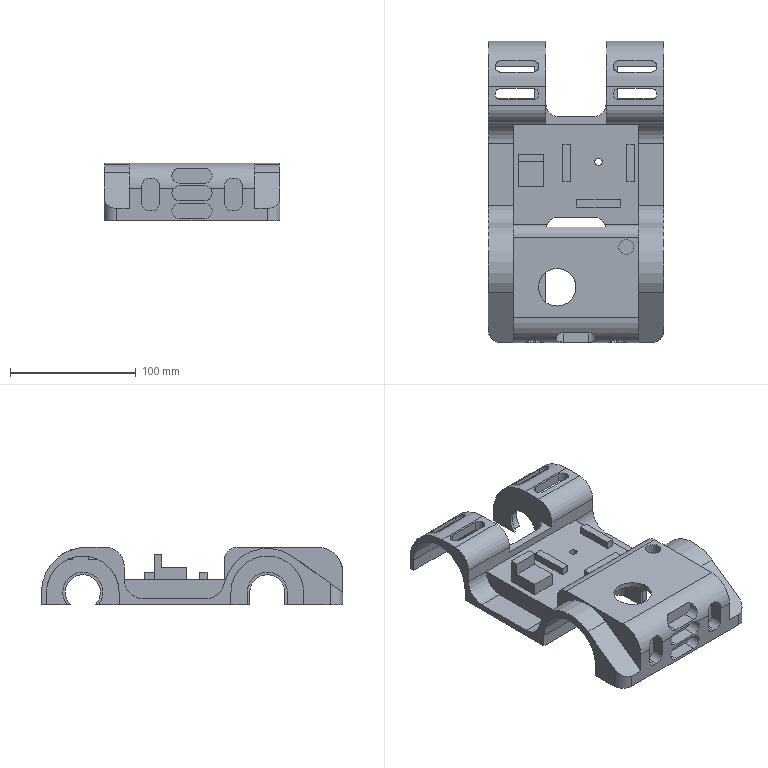Component | NX | CAR_BODY | 1 solid | 194 faces | volume 431590 mm3 | plane 125 | cylinder 69 | commonest cylinder face diameters 20 x17 12 x15 9 x8 30 x7 58 x4 28 x4 32 x4 8 x4